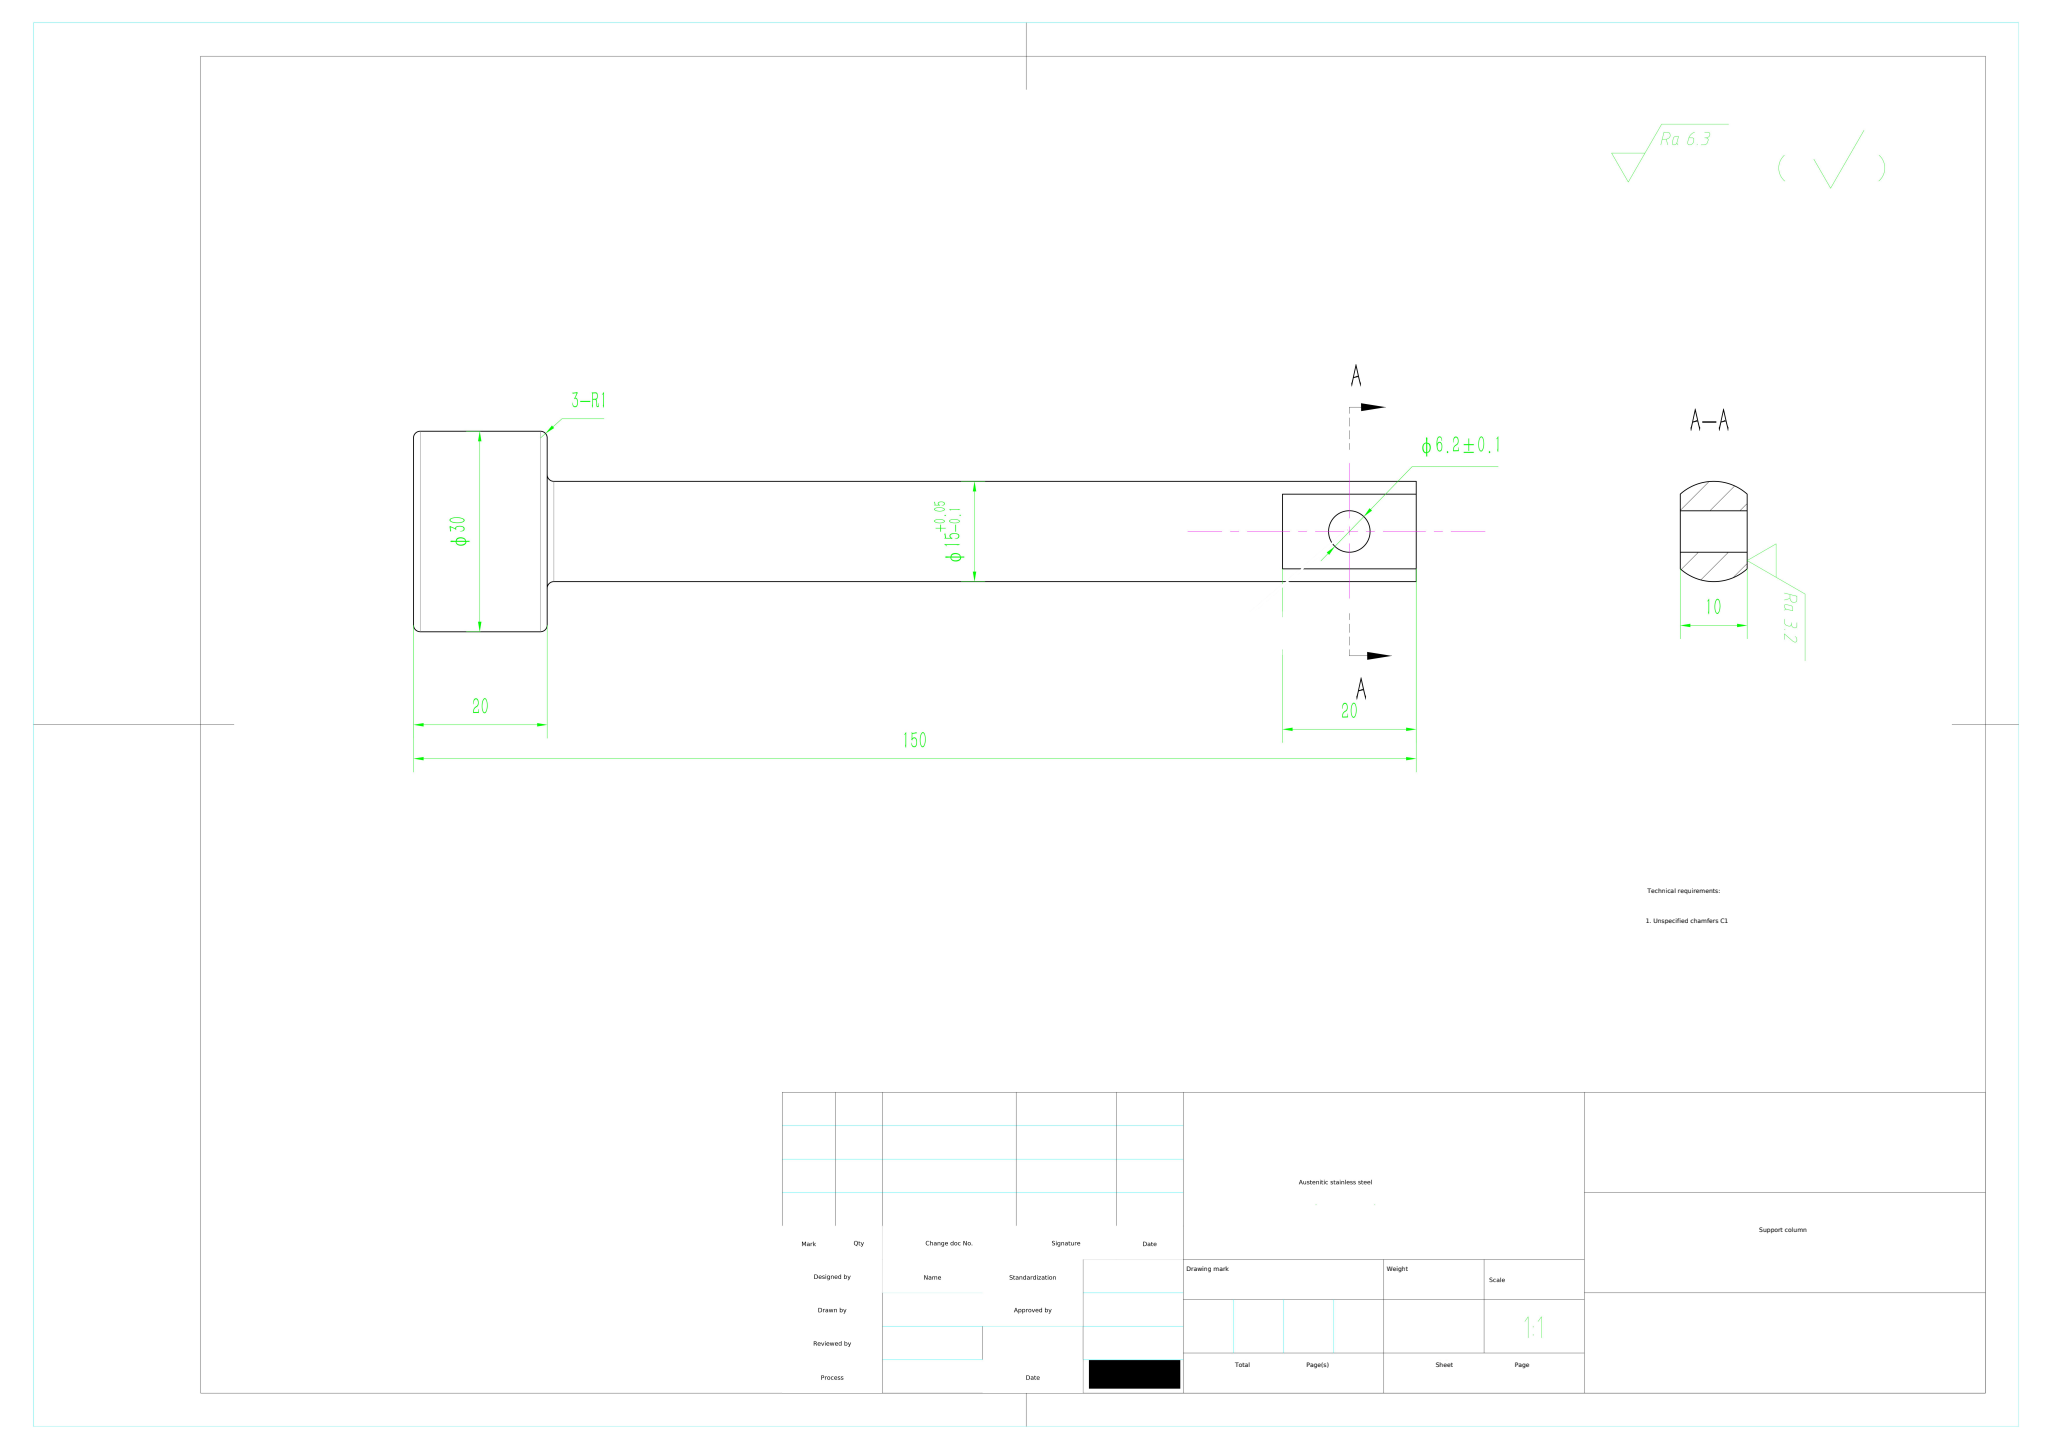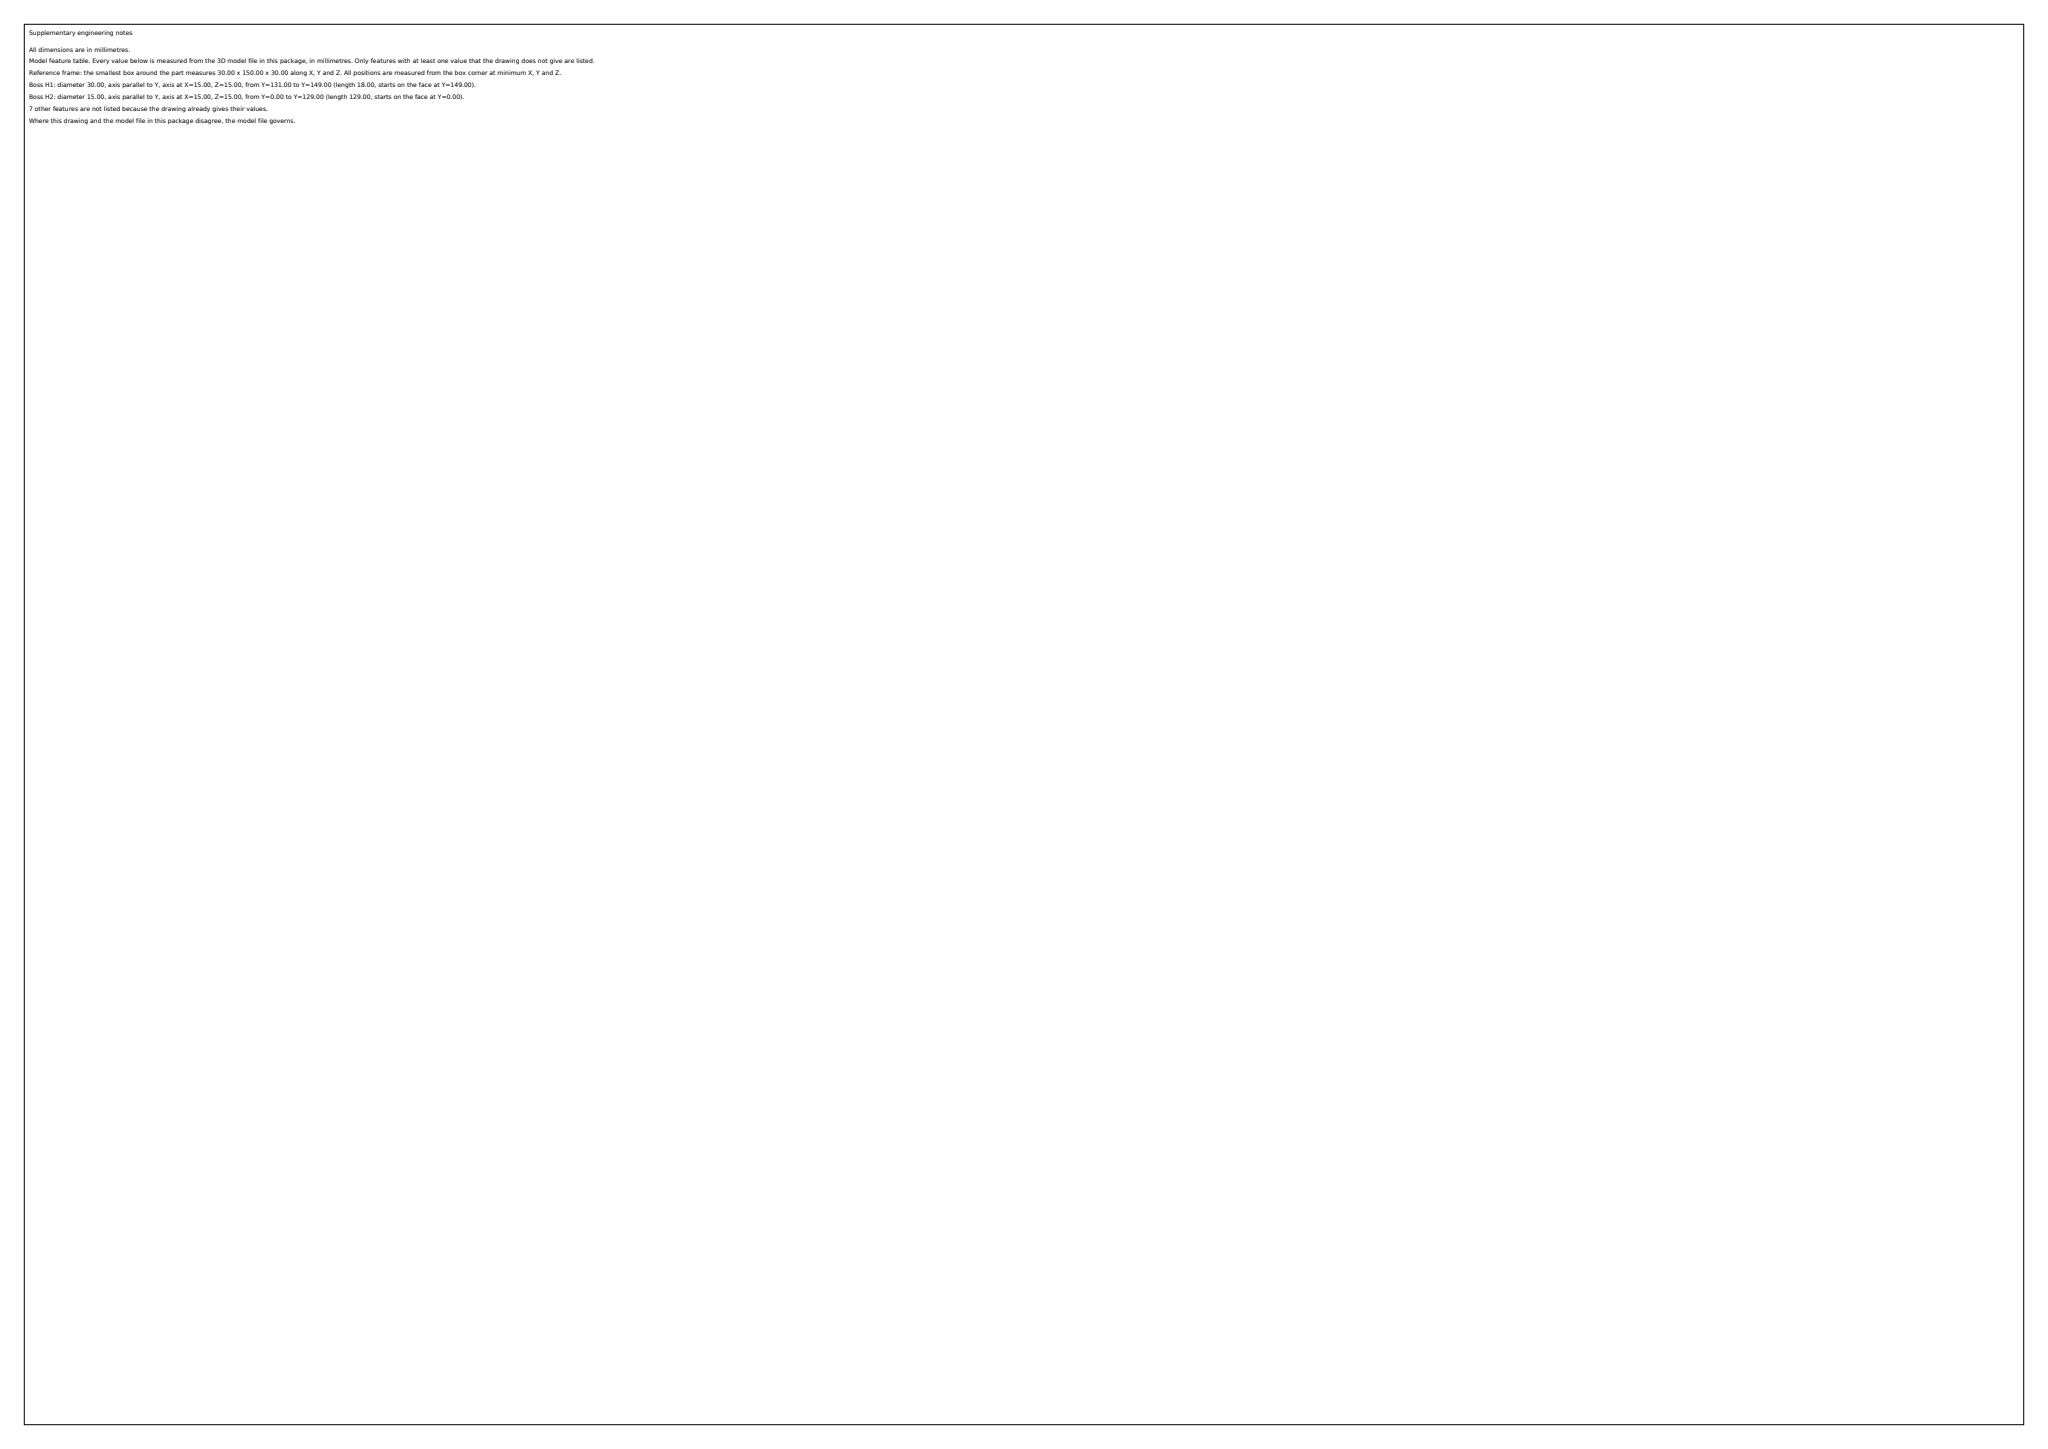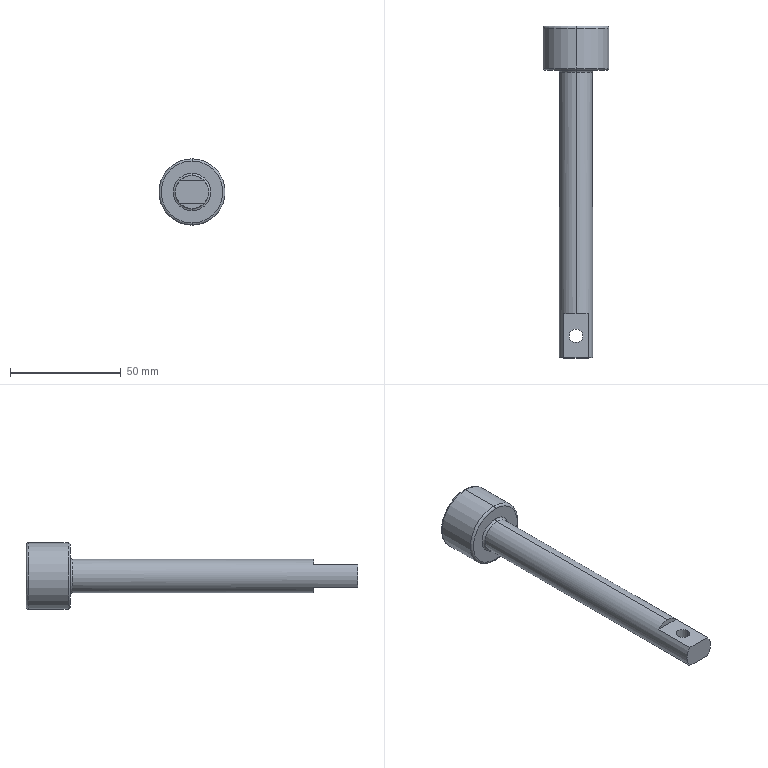Part | SolidWorks | mm | material Austenitic stainless steel | 1 solid | 19 faces | box 30 x 150 x 30 mm | volume 36004 mm3 | plane 7 | cylinder 6 | torus 6 | commonest cylinder face diameters 6.2 x2 30 x2 15 x2
STEP:
#1=CARTESIAN_POINT('',(-3.1,10.,-5.));
#2=VERTEX_POINT('',#1);
#3=CARTESIAN_POINT('',(3.1,10.,-5.));
#4=VERTEX_POINT('',#3);
#5=CARTESIAN_POINT('',(-0.,10.,-5.));
#6=DIRECTION('',(0.,0.,1.));
#7=DIRECTION('',(1.,0.,0.));
#8=AXIS2_PLACEMENT_3D('',#5,#6,#7);
#9=CIRCLE('',#8,3.1);
#10=EDGE_CURVE('',#2,#4,#9,.T.);
#11=ORIENTED_EDGE('',*,*,#10,.F.);
#12=CARTESIAN_POINT('',(-3.1,10.,5.));
#13=VERTEX_POINT('',#12);
#14=CARTESIAN_POINT('',(-3.1,10.,-15.));
#15=DIRECTION('',(0.,0.,1.));
#16=VECTOR('',#15,1000.);
#17=LINE('',#14,#16);
#18=EDGE_CURVE('',#2,#13,#17,.T.);
#19=ORIENTED_EDGE('',*,*,#18,.T.);
#20=CARTESIAN_POINT('',(3.1,10.,5.));
#21=VERTEX_POINT('',#20);
#22=CARTESIAN_POINT('',(-0.,10.,5.));
#23=DIRECTION('',(0.,0.,1.));
#24=DIRECTION('',(1.,0.,0.));
#25=AXIS2_PLACEMENT_3D('',#22,#23,#24);
#26=CIRCLE('',#25,3.1);
#27=EDGE_CURVE('',#13,#21,#26,.T.);
#28=ORIENTED_EDGE('',*,*,#27,.T.);
#29=CARTESIAN_POINT('',(3.1,10.,-15.));
#30=DIRECTION('',(0.,0.,1.));
#31=VECTOR('',#30,1000.);
#32=LINE('',#29,#31);
#33=EDGE_CURVE('',#4,#21,#32,.T.);
#34=ORIENTED_EDGE('',*,*,#33,.F.);
#35=EDGE_LOOP('',(#11,#19,#28,#34));
#36=FACE_OUTER_BOUND('',#35,.T.);
#37=CARTESIAN_POINT('',(-0.,10.,-15.));
#38=DIRECTION('',(0.,0.,1.));
#39=DIRECTION('',(1.,0.,0.));
#40=AXIS2_PLACEMENT_3D('',#37,#38,#39);
#41=CYLINDRICAL_SURFACE('',#40,3.1);
#42=ADVANCED_FACE('',(#36),#41,.F.);
#43=CARTESIAN_POINT('',(0.,130.,-14.));
#44=VERTEX_POINT('',#43);
#45=CARTESIAN_POINT('',(0.,130.,14.));
#46=VERTEX_POINT('',#45);
#47=CARTESIAN_POINT('',(0.,130.,0.));
#48=DIRECTION('',(0.,-1.,0.));
#49=DIRECTION('',(0.,0.,1.));
#50=AXIS2_PLACEMENT_3D('',#47,#48,#49);
#51=CIRCLE('',#50,14.);
#52=EDGE_CURVE('',#44,#46,#51,.T.);
#53=ORIENTED_EDGE('',*,*,#52,.F.);
#54=CARTESIAN_POINT('',(0.,131.,-15.));
#55=VERTEX_POINT('',#54);
#56=CARTESIAN_POINT('',(0.,131.,-14.));
#57=DIRECTION('',(1.,0.,0.));
#58=DIRECTION('',(0.,0.,-1.));
#59=AXIS2_PLACEMENT_3D('',#56,#57,#58);
#60=CIRCLE('',#59,1.);
#61=EDGE_CURVE('',#44,#55,#60,.T.);
#62=ORIENTED_EDGE('',*,*,#61,.T.);
#63=CARTESIAN_POINT('',(0.,131.,15.));
#64=VERTEX_POINT('',#63);
#65=CARTESIAN_POINT('',(0.,131.,0.));
#66=DIRECTION('',(0.,1.,0.));
#67=DIRECTION('',(0.,0.,1.));
#68=AXIS2_PLACEMENT_3D('',#65,#66,#67);
#69=CIRCLE('',#68,15.);
#70=EDGE_CURVE('',#64,#55,#69,.T.);
#71=ORIENTED_EDGE('',*,*,#70,.F.);
#72=CARTESIAN_POINT('',(0.,131.,14.));
#73=DIRECTION('',(-1.,0.,0.));
#74=DIRECTION('',(0.,0.,1.));
#75=AXIS2_PLACEMENT_3D('',#72,#73,#74);
#76=CIRCLE('',#75,1.);
#77=EDGE_CURVE('',#46,#64,#76,.T.);
#78=ORIENTED_EDGE('',*,*,#77,.F.);
#79=EDGE_LOOP('',(#53,#62,#71,#78));
#80=FACE_OUTER_BOUND('',#79,.T.);
#81=CARTESIAN_POINT('',(0.,131.,0.));
#82=DIRECTION('',(0.,1.,0.));
#83=DIRECTION('',(0.,0.,1.));
#84=AXIS2_PLACEMENT_3D('',#81,#82,#83);
#85=TOROIDAL_SURFACE('',#84,14.,1.);
#86=ADVANCED_FACE('',(#80),#85,.T.);
#87=CARTESIAN_POINT('',(0.,149.,-15.));
#88=VERTEX_POINT('',#87);
#89=CARTESIAN_POINT('',(0.,149.,15.));
#90=VERTEX_POINT('',#89);
#91=CARTESIAN_POINT('',(0.,149.,0.));
#92=DIRECTION('',(0.,-1.,0.));
#93=DIRECTION('',(0.,0.,1.));
#94=AXIS2_PLACEMENT_3D('',#91,#92,#93);
#95=CIRCLE('',#94,15.);
#96=EDGE_CURVE('',#88,#90,#95,.T.);
#97=ORIENTED_EDGE('',*,*,#96,.F.);
#98=CARTESIAN_POINT('',(0.,150.,-14.));
#99=VERTEX_POINT('',#98);
#100=CARTESIAN_POINT('',(0.,149.,-14.));
#101=DIRECTION('',(1.,0.,0.));
#102=DIRECTION('',(0.,0.,-1.));
#103=AXIS2_PLACEMENT_3D('',#100,#101,#102);
#104=CIRCLE('',#103,1.);
#105=EDGE_CURVE('',#88,#99,#104,.T.);
#106=ORIENTED_EDGE('',*,*,#105,.T.);
#107=CARTESIAN_POINT('',(0.,150.,14.));
#108=VERTEX_POINT('',#107);
#109=CARTESIAN_POINT('',(0.,150.,0.));
#110=DIRECTION('',(0.,1.,0.));
#111=DIRECTION('',(0.,0.,1.));
#112=AXIS2_PLACEMENT_3D('',#109,#110,#111);
#113=CIRCLE('',#112,14.);
#114=EDGE_CURVE('',#108,#99,#113,.T.);
#115=ORIENTED_EDGE('',*,*,#114,.F.);
#116=CARTESIAN_POINT('',(0.,149.,14.));
#117=DIRECTION('',(-1.,0.,0.));
#118=DIRECTION('',(0.,0.,1.));
#119=AXIS2_PLACEMENT_3D('',#116,#117,#118);
#120=CIRCLE('',#119,1.);
#121=EDGE_CURVE('',#90,#108,#120,.T.);
#122=ORIENTED_EDGE('',*,*,#121,.F.);
#123=EDGE_LOOP('',(#97,#106,#115,#122));
#124=FACE_OUTER_BOUND('',#123,.T.);
#125=CARTESIAN_POINT('',(0.,149.,0.));
#126=DIRECTION('',(0.,1.,0.));
#127=DIRECTION('',(0.,0.,1.));
#128=AXIS2_PLACEMENT_3D('',#125,#126,#127);
#129=TOROIDAL_SURFACE('',#128,14.,1.);
#130=ADVANCED_FACE('',(#124),#129,.T.);
#131=CARTESIAN_POINT('',(0.,130.,-8.5));
#132=VERTEX_POINT('',#131);
#133=CARTESIAN_POINT('',(0.,130.,8.5));
#134=VERTEX_POINT('',#133);
#135=CARTESIAN_POINT('',(0.,130.,0.));
#136=DIRECTION('',(0.,1.,0.));
#137=DIRECTION('',(0.,0.,1.));
#138=AXIS2_PLACEMENT_3D('',#135,#136,#137);
#139=CIRCLE('',#138,8.5);
#140=EDGE_CURVE('',#132,#134,#139,.T.);
#141=ORIENTED_EDGE('',*,*,#140,.F.);
#142=CARTESIAN_POINT('',(0.,129.,-7.5));
#143=VERTEX_POINT('',#142);
#144=CARTESIAN_POINT('',(0.,129.,-8.5));
#145=DIRECTION('',(1.,0.,0.));
#146=DIRECTION('',(0.,0.,-1.));
#147=AXIS2_PLACEMENT_3D('',#144,#145,#146);
#148=CIRCLE('',#147,1.);
#149=EDGE_CURVE('',#132,#143,#148,.T.);
#150=ORIENTED_EDGE('',*,*,#149,.T.);
#151=CARTESIAN_POINT('',(0.,129.,7.5));
#152=VERTEX_POINT('',#151);
#153=CARTESIAN_POINT('',(0.,129.,0.));
#154=DIRECTION('',(0.,-1.,0.));
#155=DIRECTION('',(0.,0.,1.));
#156=AXIS2_PLACEMENT_3D('',#153,#154,#155);
#157=CIRCLE('',#156,7.5);
#158=EDGE_CURVE('',#152,#143,#157,.T.);
#159=ORIENTED_EDGE('',*,*,#158,.F.);
#160=CARTESIAN_POINT('',(0.,129.,8.5));
#161=DIRECTION('',(-1.,0.,0.));
#162=DIRECTION('',(0.,0.,1.));
#163=AXIS2_PLACEMENT_3D('',#160,#161,#162);
#164=CIRCLE('',#163,1.);
#165=EDGE_CURVE('',#134,#152,#164,.T.);
#166=ORIENTED_EDGE('',*,*,#165,.F.);
#167=EDGE_LOOP('',(#141,#150,#159,#166));
#168=FACE_OUTER_BOUND('',#167,.T.);
#169=CARTESIAN_POINT('',(0.,129.,0.));
#170=DIRECTION('',(0.,1.,0.));
#171=DIRECTION('',(0.,0.,1.));
#172=AXIS2_PLACEMENT_3D('',#169,#170,#171);
#173=TOROIDAL_SURFACE('',#172,8.5,1.);
#174=ADVANCED_FACE('',(#168),#173,.F.);
#175=ORIENTED_EDGE('',*,*,#96,.T.);
#176=CARTESIAN_POINT('',(0.,150.,15.));
#177=DIRECTION('',(0.,-1.,0.));
#178=VECTOR('',#177,1000.);
#179=LINE('',#176,#178);
#180=EDGE_CURVE('',#90,#64,#179,.T.);
#181=ORIENTED_EDGE('',*,*,#180,.T.);
#182=ORIENTED_EDGE('',*,*,#70,.T.);
#183=CARTESIAN_POINT('',(0.,150.,-15.));
#184=DIRECTION('',(0.,-1.,0.));
#185=VECTOR('',#184,1000.);
#186=LINE('',#183,#185);
#187=EDGE_CURVE('',#88,#55,#186,.T.);
#188=ORIENTED_EDGE('',*,*,#187,.F.);
#189=EDGE_LOOP('',(#175,#181,#182,#188));
#190=FACE_OUTER_BOUND('',#189,.T.);
#191=CARTESIAN_POINT('',(0.,150.,0.));
#192=DIRECTION('',(0.,-1.,0.));
#193=DIRECTION('',(0.,0.,-1.));
#194=AXIS2_PLACEMENT_3D('',#191,#192,#193);
#195=CYLINDRICAL_SURFACE('',#194,15.);
#196=ADVANCED_FACE('',(#190),#195,.T.);
#197=CARTESIAN_POINT('',(0.,129.,0.));
#198=DIRECTION('',(0.,-1.,0.));
#199=DIRECTION('',(0.,0.,1.));
#200=AXIS2_PLACEMENT_3D('',#197,#198,#199);
#201=CIRCLE('',#200,7.5);
#202=EDGE_CURVE('',#143,#152,#201,.T.);
#203=ORIENTED_EDGE('',*,*,#202,.T.);
#204=CARTESIAN_POINT('',(0.,20.,7.5));
#205=VERTEX_POINT('',#204);
#206=CARTESIAN_POINT('',(0.,130.,7.5));
#207=DIRECTION('',(0.,-1.,0.));
#208=VECTOR('',#207,1000.);
#209=LINE('',#206,#208);
#210=EDGE_CURVE('',#152,#205,#209,.T.);
#211=ORIENTED_EDGE('',*,*,#210,.T.);
#212=CARTESIAN_POINT('',(5.59,20.,5.));
#213=VERTEX_POINT('',#212);
#214=CARTESIAN_POINT('',(0.,20.,0.));
#215=DIRECTION('',(0.,-1.,0.));
#216=DIRECTION('',(0.,0.,-1.));
#217=AXIS2_PLACEMENT_3D('',#214,#215,#216);
#218=CIRCLE('',#217,7.5);
#219=EDGE_CURVE('',#213,#205,#218,.T.);
#220=ORIENTED_EDGE('',*,*,#219,.F.);
#221=CARTESIAN_POINT('',(5.59,0.,5.));
#222=VERTEX_POINT('',#221);
#223=CARTESIAN_POINT('',(5.59,20.,5.));
#224=DIRECTION('',(0.,-1.,0.));
#225=VECTOR('',#224,1000.);
#226=LINE('',#223,#225);
#227=EDGE_CURVE('',#213,#222,#226,.T.);
#228=ORIENTED_EDGE('',*,*,#227,.T.);
#229=CARTESIAN_POINT('',(5.59,0.,-5.));
#230=VERTEX_POINT('',#229);
#231=CARTESIAN_POINT('',(0.,0.,0.));
#232=DIRECTION('',(0.,1.,0.));
#233=DIRECTION('',(0.,0.,1.));
#234=AXIS2_PLACEMENT_3D('',#231,#232,#233);
#235=CIRCLE('',#234,7.5);
#236=EDGE_CURVE('',#222,#230,#235,.T.);
#237=ORIENTED_EDGE('',*,*,#236,.T.);
#238=CARTESIAN_POINT('',(5.59,20.,-5.));
#239=VERTEX_POINT('',#238);
#240=CARTESIAN_POINT('',(5.59,20.,-5.));
#241=DIRECTION('',(0.,-1.,0.));
#242=VECTOR('',#241,1000.);
#243=LINE('',#240,#242);
#244=EDGE_CURVE('',#239,#230,#243,.T.);
#245=ORIENTED_EDGE('',*,*,#244,.F.);
#246=CARTESIAN_POINT('',(0.,20.,-7.5));
#247=VERTEX_POINT('',#246);
#248=CARTESIAN_POINT('',(0.,20.,0.));
#249=DIRECTION('',(0.,-1.,0.));
#250=DIRECTION('',(0.,0.,-1.));
#251=AXIS2_PLACEMENT_3D('',#248,#249,#250);
#252=CIRCLE('',#251,7.5);
#253=EDGE_CURVE('',#247,#239,#252,.T.);
#254=ORIENTED_EDGE('',*,*,#253,.F.);
#255=CARTESIAN_POINT('',(0.,130.,-7.5));
#256=DIRECTION('',(0.,-1.,0.));
#257=VECTOR('',#256,1000.);
#258=LINE('',#255,#257);
#259=EDGE_CURVE('',#143,#247,#258,.T.);
#260=ORIENTED_EDGE('',*,*,#259,.F.);
#261=EDGE_LOOP('',(#203,#211,#220,#228,#237,#245,#254,#260));
#262=FACE_OUTER_BOUND('',#261,.T.);
#263=CARTESIAN_POINT('',(0.,130.,0.));
#264=DIRECTION('',(0.,-1.,0.));
#265=DIRECTION('',(0.,0.,-1.));
#266=AXIS2_PLACEMENT_3D('',#263,#264,#265);
#267=CYLINDRICAL_SURFACE('',#266,7.5);
#268=ADVANCED_FACE('',(#262),#267,.T.);
#269=ORIENTED_EDGE('',*,*,#210,.F.);
#270=ORIENTED_EDGE('',*,*,#158,.T.);
#271=ORIENTED_EDGE('',*,*,#259,.T.);
#272=CARTESIAN_POINT('',(-5.59,20.,-5.));
#273=VERTEX_POINT('',#272);
#274=CARTESIAN_POINT('',(0.,20.,0.));
#275=DIRECTION('',(0.,-1.,0.));
#276=DIRECTION('',(0.,0.,-1.));
#277=AXIS2_PLACEMENT_3D('',#274,#275,#276);
#278=CIRCLE('',#277,7.5);
#279=EDGE_CURVE('',#273,#247,#278,.T.);
#280=ORIENTED_EDGE('',*,*,#279,.F.);
#281=CARTESIAN_POINT('',(-5.59,0.,-5.));
#282=VERTEX_POINT('',#281);
#283=CARTESIAN_POINT('',(-5.59,20.,-5.));
#284=DIRECTION('',(0.,-1.,0.));
#285=VECTOR('',#284,1000.);
#286=LINE('',#283,#285);
#287=EDGE_CURVE('',#273,#282,#286,.T.);
#288=ORIENTED_EDGE('',*,*,#287,.T.);
#289=CARTESIAN_POINT('',(-5.59,0.,5.));
#290=VERTEX_POINT('',#289);
#291=CARTESIAN_POINT('',(0.,0.,0.));
#292=DIRECTION('',(0.,1.,0.));
#293=DIRECTION('',(0.,0.,1.));
#294=AXIS2_PLACEMENT_3D('',#291,#292,#293);
#295=CIRCLE('',#294,7.5);
#296=EDGE_CURVE('',#282,#290,#295,.T.);
#297=ORIENTED_EDGE('',*,*,#296,.T.);
#298=CARTESIAN_POINT('',(-5.59,20.,5.));
#299=VERTEX_POINT('',#298);
#300=CARTESIAN_POINT('',(-5.59,20.,5.));
#301=DIRECTION('',(0.,-1.,0.));
#302=VECTOR('',#301,1000.);
#303=LINE('',#300,#302);
#304=EDGE_CURVE('',#299,#290,#303,.T.);
#305=ORIENTED_EDGE('',*,*,#304,.F.);
#306=CARTESIAN_POINT('',(0.,20.,0.));
#307=DIRECTION('',(0.,-1.,0.));
#308=DIRECTION('',(0.,0.,-1.));
#309=AXIS2_PLACEMENT_3D('',#306,#307,#308);
#310=CIRCLE('',#309,7.5);
#311=EDGE_CURVE('',#205,#299,#310,.T.);
#312=ORIENTED_EDGE('',*,*,#311,.F.);
#313=EDGE_LOOP('',(#269,#270,#271,#280,#288,#297,#305,#312));
#314=FACE_OUTER_BOUND('',#313,.T.);
#315=CARTESIAN_POINT('',(0.,130.,0.));
#316=DIRECTION('',(0.,-1.,0.));
#317=DIRECTION('',(0.,0.,-1.));
#318=AXIS2_PLACEMENT_3D('',#315,#316,#317);
#319=CYLINDRICAL_SURFACE('',#318,7.5);
#320=ADVANCED_FACE('',(#314),#319,.T.);
#321=ORIENTED_EDGE('',*,*,#296,.F.);
#322=CARTESIAN_POINT('',(-5.59,0.,-5.));
#323=DIRECTION('',(-1.,0.,0.));
#324=VECTOR('',#323,1000.);
#325=LINE('',#322,#324);
#326=EDGE_CURVE('',#230,#282,#325,.T.);
#327=ORIENTED_EDGE('',*,*,#326,.F.);
#328=ORIENTED_EDGE('',*,*,#236,.F.);
#329=CARTESIAN_POINT('',(-5.59,0.,5.));
#330=DIRECTION('',(1.,0.,0.));
#331=VECTOR('',#330,1000.);
#332=LINE('',#329,#331);
#333=EDGE_CURVE('',#290,#222,#332,.T.);
#334=ORIENTED_EDGE('',*,*,#333,.F.);
#335=EDGE_LOOP('',(#321,#327,#328,#334));
#336=FACE_OUTER_BOUND('',#335,.T.);
#337=CARTESIAN_POINT('',(0.,0.,0.));
#338=DIRECTION('',(0.,1.,0.));
#339=DIRECTION('',(0.,0.,1.));
#340=AXIS2_PLACEMENT_3D('',#337,#338,#339);
#341=PLANE('',#340);
#342=ADVANCED_FACE('',(#336),#341,.F.);
#343=ORIENTED_EDGE('',*,*,#180,.F.);
#344=CARTESIAN_POINT('',(0.,149.,0.));
#345=DIRECTION('',(0.,-1.,0.));
#346=DIRECTION('',(0.,0.,1.));
#347=AXIS2_PLACEMENT_3D('',#344,#345,#346);
#348=CIRCLE('',#347,15.);
#349=EDGE_CURVE('',#90,#88,#348,.T.);
#350=ORIENTED_EDGE('',*,*,#349,.T.);
#351=ORIENTED_EDGE('',*,*,#187,.T.);
#352=CARTESIAN_POINT('',(0.,131.,0.));
#353=DIRECTION('',(0.,1.,0.));
#354=DIRECTION('',(0.,0.,1.));
#355=AXIS2_PLACEMENT_3D('',#352,#353,#354);
#356=CIRCLE('',#355,15.);
#357=EDGE_CURVE('',#55,#64,#356,.T.);
#358=ORIENTED_EDGE('',*,*,#357,.T.);
#359=EDGE_LOOP('',(#343,#350,#351,#358));
#360=FACE_OUTER_BOUND('',#359,.T.);
#361=CARTESIAN_POINT('',(0.,150.,0.));
#362=DIRECTION('',(0.,-1.,0.));
#363=DIRECTION('',(0.,0.,-1.));
#364=AXIS2_PLACEMENT_3D('',#361,#362,#363);
#365=CYLINDRICAL_SURFACE('',#364,15.);
#366=ADVANCED_FACE('',(#360),#365,.T.);
#367=ORIENTED_EDGE('',*,*,#114,.T.);
#368=CARTESIAN_POINT('',(0.,150.,0.));
#369=DIRECTION('',(0.,1.,0.));
#370=DIRECTION('',(0.,0.,1.));
#371=AXIS2_PLACEMENT_3D('',#368,#369,#370);
#372=CIRCLE('',#371,14.);
#373=EDGE_CURVE('',#99,#108,#372,.T.);
#374=ORIENTED_EDGE('',*,*,#373,.T.);
#375=EDGE_LOOP('',(#367,#374));
#376=FACE_OUTER_BOUND('',#375,.T.);
#377=CARTESIAN_POINT('',(0.,150.,0.));
#378=DIRECTION('',(0.,1.,0.));
#379=DIRECTION('',(0.,0.,1.));
#380=AXIS2_PLACEMENT_3D('',#377,#378,#379);
#381=PLANE('',#380);
#382=ADVANCED_FACE('',(#376),#381,.T.);
#383=CARTESIAN_POINT('',(0.,130.,0.));
#384=DIRECTION('',(0.,1.,0.));
#385=DIRECTION('',(0.,0.,1.));
#386=AXIS2_PLACEMENT_3D('',#383,#384,#385);
#387=CIRCLE('',#386,8.5);
#388=EDGE_CURVE('',#134,#132,#387,.T.);
#389=ORIENTED_EDGE('',*,*,#388,.T.);
#390=ORIENTED_EDGE('',*,*,#140,.T.);
#391=EDGE_LOOP('',(#389,#390));
#392=FACE_BOUND('',#391,.T.);
#393=CARTESIAN_POINT('',(0.,130.,0.));
#394=DIRECTION('',(0.,-1.,0.));
#395=DIRECTION('',(0.,0.,1.));
#396=AXIS2_PLACEMENT_3D('',#393,#394,#395);
#397=CIRCLE('',#396,14.);
#398=EDGE_CURVE('',#46,#44,#397,.T.);
#399=ORIENTED_EDGE('',*,*,#398,.T.);
#400=ORIENTED_EDGE('',*,*,#52,.T.);
#401=EDGE_LOOP('',(#399,#400));
#402=FACE_OUTER_BOUND('',#401,.T.);
#403=CARTESIAN_POINT('',(0.,130.,0.));
#404=DIRECTION('',(0.,1.,0.));
#405=DIRECTION('',(0.,0.,1.));
#406=AXIS2_PLACEMENT_3D('',#403,#404,#405);
#407=PLANE('',#406);
#408=ADVANCED_FACE('',(#392,#402),#407,.F.);
#409=ORIENTED_EDGE('',*,*,#149,.F.);
#410=ORIENTED_EDGE('',*,*,#388,.F.);
#411=ORIENTED_EDGE('',*,*,#165,.T.);
#412=ORIENTED_EDGE('',*,*,#202,.F.);
#413=EDGE_LOOP('',(#409,#410,#411,#412));
#414=FACE_OUTER_BOUND('',#413,.T.);
#415=CARTESIAN_POINT('',(0.,129.,0.));
#416=DIRECTION('',(0.,1.,0.));
#417=DIRECTION('',(0.,0.,1.));
#418=AXIS2_PLACEMENT_3D('',#415,#416,#417);
#419=TOROIDAL_SURFACE('',#418,8.5,1.);
#420=ADVANCED_FACE('',(#414),#419,.F.);
#421=ORIENTED_EDGE('',*,*,#105,.F.);
#422=ORIENTED_EDGE('',*,*,#349,.F.);
#423=ORIENTED_EDGE('',*,*,#121,.T.);
#424=ORIENTED_EDGE('',*,*,#373,.F.);
#425=EDGE_LOOP('',(#421,#422,#423,#424));
#426=FACE_OUTER_BOUND('',#425,.T.);
#427=CARTESIAN_POINT('',(0.,149.,0.));
#428=DIRECTION('',(0.,1.,0.));
#429=DIRECTION('',(0.,0.,1.));
#430=AXIS2_PLACEMENT_3D('',#427,#428,#429);
#431=TOROIDAL_SURFACE('',#430,14.,1.);
#432=ADVANCED_FACE('',(#426),#431,.T.);
#433=ORIENTED_EDGE('',*,*,#61,.F.);
#434=ORIENTED_EDGE('',*,*,#398,.F.);
#435=ORIENTED_EDGE('',*,*,#77,.T.);
#436=ORIENTED_EDGE('',*,*,#357,.F.);
#437=EDGE_LOOP('',(#433,#434,#435,#436));
#438=FACE_OUTER_BOUND('',#437,.T.);
#439=CARTESIAN_POINT('',(0.,131.,0.));
#440=DIRECTION('',(0.,1.,0.));
#441=DIRECTION('',(0.,0.,1.));
#442=AXIS2_PLACEMENT_3D('',#439,#440,#441);
#443=TOROIDAL_SURFACE('',#442,14.,1.);
#444=ADVANCED_FACE('',(#438),#443,.T.);
#445=CARTESIAN_POINT('',(-0.,10.,5.));
#446=DIRECTION('',(0.,0.,1.));
#447=DIRECTION('',(1.,0.,0.));
#448=AXIS2_PLACEMENT_3D('',#445,#446,#447);
#449=CIRCLE('',#448,3.1);
#450=EDGE_CURVE('',#21,#13,#449,.T.);
#451=ORIENTED_EDGE('',*,*,#450,.F.);
#452=ORIENTED_EDGE('',*,*,#27,.F.);
#453=EDGE_LOOP('',(#451,#452));
#454=FACE_BOUND('',#453,.T.);
#455=ORIENTED_EDGE('',*,*,#333,.T.);
#456=ORIENTED_EDGE('',*,*,#227,.F.);
#457=CARTESIAN_POINT('',(-5.59,20.,5.));
#458=DIRECTION('',(1.,0.,0.));
#459=VECTOR('',#458,1000.);
#460=LINE('',#457,#459);
#461=EDGE_CURVE('',#299,#213,#460,.T.);
#462=ORIENTED_EDGE('',*,*,#461,.F.);
#463=ORIENTED_EDGE('',*,*,#304,.T.);
#464=EDGE_LOOP('',(#455,#456,#462,#463));
#465=FACE_OUTER_BOUND('',#464,.T.);
#466=CARTESIAN_POINT('',(-5.59,20.,5.));
#467=DIRECTION('',(0.,0.,-1.));
#468=DIRECTION('',(-1.,0.,0.));
#469=AXIS2_PLACEMENT_3D('',#466,#467,#468);
#470=PLANE('',#469);
#471=ADVANCED_FACE('',(#454,#465),#470,.F.);
#472=ORIENTED_EDGE('',*,*,#219,.T.);
#473=ORIENTED_EDGE('',*,*,#311,.T.);
#474=ORIENTED_EDGE('',*,*,#461,.T.);
#475=EDGE_LOOP('',(#472,#473,#474));
#476=FACE_OUTER_BOUND('',#475,.T.);
#477=CARTESIAN_POINT('',(0.,20.,0.));
#478=DIRECTION('',(0.,-1.,0.));
#479=DIRECTION('',(0.,0.,-1.));
#480=AXIS2_PLACEMENT_3D('',#477,#478,#479);
#481=PLANE('',#480);
#482=ADVANCED_FACE('',(#476),#481,.T.);
#483=CARTESIAN_POINT('',(-0.,10.,-5.));
#484=DIRECTION('',(0.,0.,1.));
#485=DIRECTION('',(1.,0.,0.));
#486=AXIS2_PLACEMENT_3D('',#483,#484,#485);
#487=CIRCLE('',#486,3.1);
#488=EDGE_CURVE('',#4,#2,#487,.T.);
#489=ORIENTED_EDGE('',*,*,#488,.T.);
#490=ORIENTED_EDGE('',*,*,#10,.T.);
#491=EDGE_LOOP('',(#489,#490));
#492=FACE_BOUND('',#491,.T.);
#493=ORIENTED_EDGE('',*,*,#326,.T.);
#494=ORIENTED_EDGE('',*,*,#287,.F.);
#495=CARTESIAN_POINT('',(-5.59,20.,-5.));
#496=DIRECTION('',(-1.,0.,0.));
#497=VECTOR('',#496,1000.);
#498=LINE('',#495,#497);
#499=EDGE_CURVE('',#239,#273,#498,.T.);
#500=ORIENTED_EDGE('',*,*,#499,.F.);
#501=ORIENTED_EDGE('',*,*,#244,.T.);
#502=EDGE_LOOP('',(#493,#494,#500,#501));
#503=FACE_OUTER_BOUND('',#502,.T.);
#504=CARTESIAN_POINT('',(-5.59,20.,-5.));
#505=DIRECTION('',(0.,0.,1.));
#506=DIRECTION('',(1.,0.,0.));
#507=AXIS2_PLACEMENT_3D('',#504,#505,#506);
#508=PLANE('',#507);
#509=ADVANCED_FACE('',(#492,#503),#508,.F.);
#510=ORIENTED_EDGE('',*,*,#279,.T.);
#511=ORIENTED_EDGE('',*,*,#253,.T.);
#512=ORIENTED_EDGE('',*,*,#499,.T.);
#513=EDGE_LOOP('',(#510,#511,#512));
#514=FACE_OUTER_BOUND('',#513,.T.);
#515=CARTESIAN_POINT('',(0.,20.,0.));
#516=DIRECTION('',(0.,-1.,0.));
#517=DIRECTION('',(0.,0.,-1.));
#518=AXIS2_PLACEMENT_3D('',#515,#516,#517);
#519=PLANE('',#518);
#520=ADVANCED_FACE('',(#514),#519,.T.);
#521=ORIENTED_EDGE('',*,*,#18,.F.);
#522=ORIENTED_EDGE('',*,*,#488,.F.);
#523=ORIENTED_EDGE('',*,*,#33,.T.);
#524=ORIENTED_EDGE('',*,*,#450,.T.);
#525=EDGE_LOOP('',(#521,#522,#523,#524));
#526=FACE_OUTER_BOUND('',#525,.T.);
#527=CARTESIAN_POINT('',(-0.,10.,-15.));
#528=DIRECTION('',(0.,0.,1.));
#529=DIRECTION('',(1.,0.,0.));
#530=AXIS2_PLACEMENT_3D('',#527,#528,#529);
#531=CYLINDRICAL_SURFACE('',#530,3.1);
#532=ADVANCED_FACE('',(#526),#531,.F.);
#533=CLOSED_SHELL('',(#42,#86,#130,#174,#196,#268,#320,#342,#366,#382,#408,#420,#432,#444,#471,#482,#509,#520,#532));
#534=MANIFOLD_SOLID_BREP('',#533);
#535=CARTESIAN_POINT('',(0.,0.,0.));
#536=DIRECTION('',(0.,0.,1.));
#537=DIRECTION('',(1.,0.,0.));
#538=AXIS2_PLACEMENT_3D('',#535,#536,#537);
#539=(LENGTH_UNIT()NAMED_UNIT(*)SI_UNIT(.MILLI.,.METRE.));
#540=UNCERTAINTY_MEASURE_WITH_UNIT(LENGTH_MEASURE(0.00001),#539,'','');
#541=(NAMED_UNIT(*)PLANE_ANGLE_UNIT()SI_UNIT($,.RADIAN.));
#542=(NAMED_UNIT(*)SI_UNIT($,.STERADIAN.)SOLID_ANGLE_UNIT());
#543=(GEOMETRIC_REPRESENTATION_CONTEXT(3)GLOBAL_UNCERTAINTY_ASSIGNED_CONTEXT((#540))GLOBAL_UNIT_ASSIGNED_CONTEXT((#539,#541,#542))REPRESENTATION_CONTEXT('',''));
#544=ADVANCED_BREP_SHAPE_REPRESENTATION('',(#534,#538),#543);